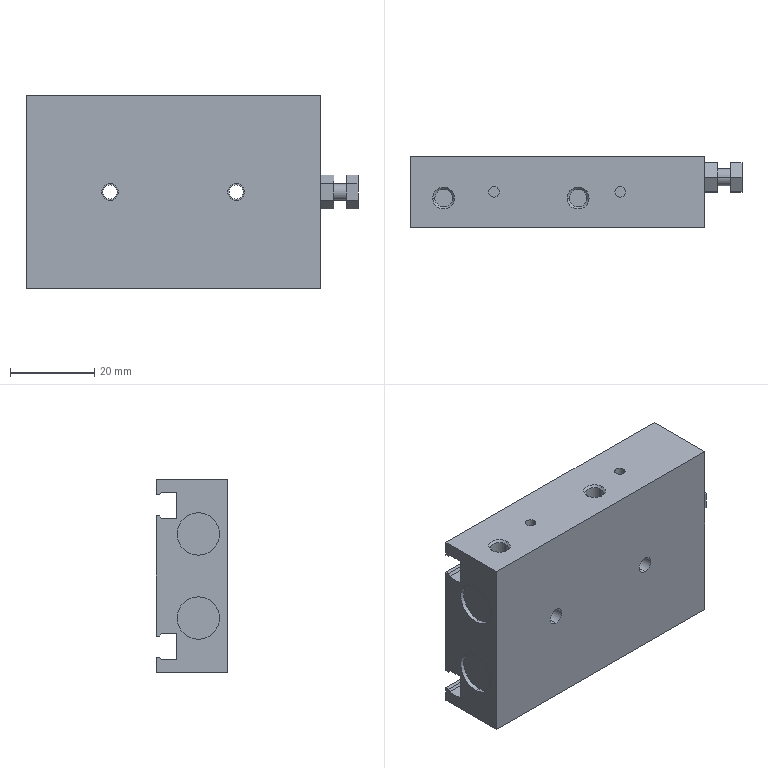Component | SolidWorks | F-YBExport-1-1_F-YBXCXSM10-15-Z73L-1_F-YBXCXSM10-15-Z73L_cyl_cxs(CXS10-15)-1 | 1 solid | 105 faces | volume 46168 mm3 | plane 55 | cylinder 42 | cone 8 | commonest cylinder face diameters 10.1 x8 2.5 x8 4.2 x8 4 x6 6.5 x4 6.1 x4 3.4 x4